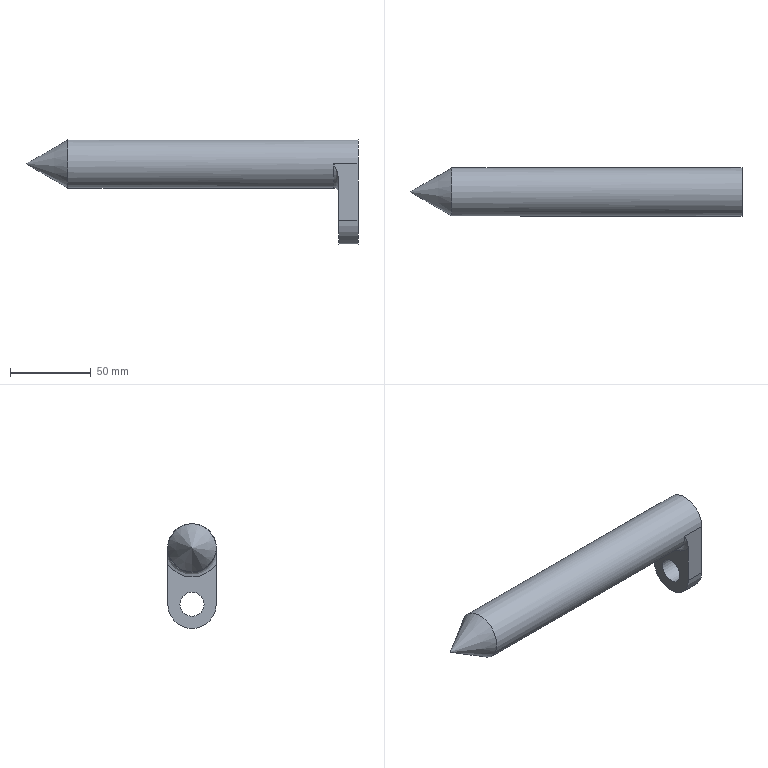Component | NX | CENTRE_HEAD2 | 1 solid | 9 faces | box 205.98 x 30 x 65 mm | volume 143914 mm3 | plane 4 | cylinder 3 | cone 1 | torus 1 | commonest cylinder face diameters 30 x2 15 x1
STEP:
#1=CARTESIAN_POINT('',(0.,0.,0.));
#2=DIRECTION('',(0.,0.,1.));
#3=DIRECTION('',(1.,0.,0.));
#4=AXIS2_PLACEMENT_3D('',#1,#2,#3);
#5=CARTESIAN_POINT('',(157.,15.,137.5));
#6=VERTEX_POINT('',#5);
#7=CARTESIAN_POINT('',(157.,-15.,137.5));
#8=VERTEX_POINT('',#7);
#9=CARTESIAN_POINT('',(157.,0.,137.5));
#10=DIRECTION('',(1.,0.,0.));
#11=DIRECTION('',(0.,0.,-1.));
#12=AXIS2_PLACEMENT_3D('',#9,#10,#11);
#13=CIRCLE('',#12,15.);
#14=CARTESIAN_POINT('',(157.,0.,137.5));
#15=DIRECTION('',(1.,0.,0.));
#16=DIRECTION('',(0.,0.,-1.));
#17=AXIS2_PLACEMENT_3D('',#14,#15,#16);
#18=PLANE('',#17);
#19=CARTESIAN_POINT('',(0.,0.));
#20=DIRECTION('',(1.,0.));
#21=AXIS2_PLACEMENT_2D('',#19,#20);
#22=CIRCLE('',#21,15.);
#23=(GEOMETRIC_REPRESENTATION_CONTEXT(2)PARAMETRIC_REPRESENTATION_CONTEXT()REPRESENTATION_CONTEXT('',''));
#24=DEFINITIONAL_REPRESENTATION('',(#22),#23);
#25=PCURVE('',#18,#24);
#26=CARTESIAN_POINT('',(-48.981,0.,137.5));
#27=DIRECTION('',(1.,0.,0.));
#28=DIRECTION('',(0.,0.,-1.));
#29=AXIS2_PLACEMENT_3D('',#26,#27,#28);
#30=CYLINDRICAL_SURFACE('',#29,15.);
#31=CARTESIAN_POINT('',(0.,205.981));
#32=DIRECTION('',(1.,0.));
#33=VECTOR('',#32,1.);
#34=LINE('',#31,#33);
#35=(GEOMETRIC_REPRESENTATION_CONTEXT(2)PARAMETRIC_REPRESENTATION_CONTEXT()REPRESENTATION_CONTEXT('',''));
#36=DEFINITIONAL_REPRESENTATION('',(#34),#35);
#37=PCURVE('',#30,#36);
#38=SURFACE_CURVE('',#13,(#25,#37),.PCURVE_S1.);
#39=EDGE_CURVE('',#6,#8,#38,.T.);
#40=ORIENTED_EDGE('',*,*,#39,.T.);
#41=CARTESIAN_POINT('',(157.,-15.,102.5));
#42=VERTEX_POINT('',#41);
#43=CARTESIAN_POINT('',(157.,-15.,102.5));
#44=DIRECTION('',(0.,0.,1.));
#45=VECTOR('',#44,1.);
#46=LINE('',#43,#45);
#47=CARTESIAN_POINT('',(35.,-15.));
#48=DIRECTION('',(-1.,0.));
#49=VECTOR('',#48,1.);
#50=LINE('',#47,#49);
#51=(GEOMETRIC_REPRESENTATION_CONTEXT(2)PARAMETRIC_REPRESENTATION_CONTEXT()REPRESENTATION_CONTEXT('',''));
#52=DEFINITIONAL_REPRESENTATION('',(#50),#51);
#53=PCURVE('',#18,#52);
#54=CARTESIAN_POINT('',(145.,-15.,102.5));
#55=DIRECTION('',(0.,1.,-0.));
#56=DIRECTION('',(0.,0.,1.));
#57=AXIS2_PLACEMENT_3D('',#54,#55,#56);
#58=PLANE('',#57);
#59=CARTESIAN_POINT('',(0.,12.));
#60=DIRECTION('',(1.,0.));
#61=VECTOR('',#60,1.);
#62=LINE('',#59,#61);
#63=(GEOMETRIC_REPRESENTATION_CONTEXT(2)PARAMETRIC_REPRESENTATION_CONTEXT()REPRESENTATION_CONTEXT('',''));
#64=DEFINITIONAL_REPRESENTATION('',(#62),#63);
#65=PCURVE('',#58,#64);
#66=SURFACE_CURVE('',#46,(#53,#65),.PCURVE_S1.);
#67=EDGE_CURVE('',#42,#8,#66,.T.);
#68=ORIENTED_EDGE('',*,*,#67,.F.);
#69=CARTESIAN_POINT('',(157.,15.,102.5));
#70=VERTEX_POINT('',#69);
#71=CARTESIAN_POINT('',(157.,0.,102.5));
#72=DIRECTION('',(-1.,0.,0.));
#73=DIRECTION('',(0.,1.,0.));
#74=AXIS2_PLACEMENT_3D('',#71,#72,#73);
#75=CIRCLE('',#74,15.);
#76=CARTESIAN_POINT('',(35.,15.));
#77=CARTESIAN_POINT('',(60.981,15.));
#78=CARTESIAN_POINT('',(47.99,-7.5));
#79=CARTESIAN_POINT('',(35.,-30.));
#80=CARTESIAN_POINT('',(22.01,-7.5));
#81=CARTESIAN_POINT('',(9.019,15.));
#82=CARTESIAN_POINT('',(35.,15.));
#83=(BOUNDED_CURVE()B_SPLINE_CURVE(2,(#76,#77,#78,#79,#80,#81,#82),.UNSPECIFIED.,.T.,.F.)B_SPLINE_CURVE_WITH_KNOTS((1,2,2,2,2,1),(-2.094,0.,2.094,4.189,6.283,8.378),.UNSPECIFIED.)CURVE()GEOMETRIC_REPRESENTATION_ITEM()RATIONAL_B_SPLINE_CURVE((1.,0.5,1.,0.5,1.,0.5,1.))REPRESENTATION_ITEM(''));
#84=(GEOMETRIC_REPRESENTATION_CONTEXT(2)PARAMETRIC_REPRESENTATION_CONTEXT()REPRESENTATION_CONTEXT('',''));
#85=DEFINITIONAL_REPRESENTATION('',(#83),#84);
#86=PCURVE('',#18,#85);
#87=CARTESIAN_POINT('',(145.,0.,102.5));
#88=DIRECTION('',(1.,0.,0.));
#89=DIRECTION('',(0.,0.,-1.));
#90=AXIS2_PLACEMENT_3D('',#87,#88,#89);
#91=CYLINDRICAL_SURFACE('',#90,15.);
#92=CARTESIAN_POINT('',(1.571,12.));
#93=DIRECTION('',(-1.,0.));
#94=VECTOR('',#93,1.);
#95=LINE('',#92,#94);
#96=(GEOMETRIC_REPRESENTATION_CONTEXT(2)PARAMETRIC_REPRESENTATION_CONTEXT()REPRESENTATION_CONTEXT('',''));
#97=DEFINITIONAL_REPRESENTATION('',(#95),#96);
#98=PCURVE('',#91,#97);
#99=SURFACE_CURVE('',#75,(#86,#98),.PCURVE_S1.);
#100=EDGE_CURVE('',#70,#42,#99,.T.);
#101=ORIENTED_EDGE('',*,*,#100,.F.);
#102=CARTESIAN_POINT('',(157.,15.,137.5));
#103=DIRECTION('',(0.,0.,-1.));
#104=VECTOR('',#103,1.);
#105=LINE('',#102,#104);
#106=CARTESIAN_POINT('',(0.,15.));
#107=DIRECTION('',(1.,0.));
#108=VECTOR('',#107,1.);
#109=LINE('',#106,#108);
#110=(GEOMETRIC_REPRESENTATION_CONTEXT(2)PARAMETRIC_REPRESENTATION_CONTEXT()REPRESENTATION_CONTEXT('',''));
#111=DEFINITIONAL_REPRESENTATION('',(#109),#110);
#112=PCURVE('',#18,#111);
#113=CARTESIAN_POINT('',(145.,15.,137.5));
#114=DIRECTION('',(0.,-1.,0.));
#115=DIRECTION('',(0.,0.,-1.));
#116=AXIS2_PLACEMENT_3D('',#113,#114,#115);
#117=PLANE('',#116);
#118=CARTESIAN_POINT('',(0.,12.));
#119=DIRECTION('',(1.,0.));
#120=VECTOR('',#119,1.);
#121=LINE('',#118,#120);
#122=(GEOMETRIC_REPRESENTATION_CONTEXT(2)PARAMETRIC_REPRESENTATION_CONTEXT()REPRESENTATION_CONTEXT('',''));
#123=DEFINITIONAL_REPRESENTATION('',(#121),#122);
#124=PCURVE('',#117,#123);
#125=SURFACE_CURVE('',#105,(#112,#124),.PCURVE_S1.);
#126=EDGE_CURVE('',#6,#70,#125,.T.);
#127=ORIENTED_EDGE('',*,*,#126,.F.);
#128=EDGE_LOOP('',(#40,#68,#101,#127));
#129=FACE_BOUND('',#128,.T.);
#130=CARTESIAN_POINT('',(157.,7.5,102.5));
#131=VERTEX_POINT('',#130);
#132=CARTESIAN_POINT('',(157.,0.,102.5));
#133=DIRECTION('',(-1.,0.,0.));
#134=DIRECTION('',(0.,1.,0.));
#135=AXIS2_PLACEMENT_3D('',#132,#133,#134);
#136=CIRCLE('',#135,7.5);
#137=CARTESIAN_POINT('',(35.,7.5));
#138=CARTESIAN_POINT('',(47.99,7.5));
#139=CARTESIAN_POINT('',(41.495,-3.75));
#140=CARTESIAN_POINT('',(35.,-15.));
#141=CARTESIAN_POINT('',(28.505,-3.75));
#142=CARTESIAN_POINT('',(22.01,7.5));
#143=CARTESIAN_POINT('',(35.,7.5));
#144=(BOUNDED_CURVE()B_SPLINE_CURVE(2,(#137,#138,#139,#140,#141,#142,#143),.UNSPECIFIED.,.T.,.F.)B_SPLINE_CURVE_WITH_KNOTS((1,2,2,2,2,1),(-2.094,0.,2.094,4.189,6.283,8.378),.UNSPECIFIED.)CURVE()GEOMETRIC_REPRESENTATION_ITEM()RATIONAL_B_SPLINE_CURVE((1.,0.5,1.,0.5,1.,0.5,1.))REPRESENTATION_ITEM(''));
#145=(GEOMETRIC_REPRESENTATION_CONTEXT(2)PARAMETRIC_REPRESENTATION_CONTEXT()REPRESENTATION_CONTEXT('',''));
#146=DEFINITIONAL_REPRESENTATION('',(#144),#145);
#147=PCURVE('',#18,#146);
#148=CARTESIAN_POINT('',(145.,0.,102.5));
#149=DIRECTION('',(1.,0.,0.));
#150=DIRECTION('',(0.,0.,-1.));
#151=AXIS2_PLACEMENT_3D('',#148,#149,#150);
#152=CYLINDRICAL_SURFACE('',#151,7.5);
#153=CARTESIAN_POINT('',(7.854,12.));
#154=DIRECTION('',(-1.,0.));
#155=VECTOR('',#154,1.);
#156=LINE('',#153,#155);
#157=(GEOMETRIC_REPRESENTATION_CONTEXT(2)PARAMETRIC_REPRESENTATION_CONTEXT()REPRESENTATION_CONTEXT('',''));
#158=DEFINITIONAL_REPRESENTATION('',(#156),#157);
#159=PCURVE('',#152,#158);
#160=SURFACE_CURVE('',#136,(#147,#159),.PCURVE_S1.);
#161=EDGE_CURVE('',#131,#131,#160,.T.);
#162=ORIENTED_EDGE('',*,*,#161,.T.);
#163=EDGE_LOOP('',(#162));
#164=FACE_BOUND('',#163,.T.);
#165=ADVANCED_FACE('',(#129,#164),#18,.T.);
#166=CARTESIAN_POINT('',(-48.981,0.,137.5));
#167=VERTEX_POINT('',#166);
#168=CARTESIAN_POINT('',(-23.,0.,122.5));
#169=VERTEX_POINT('',#168);
#170=CARTESIAN_POINT('',(-48.981,0.,137.5));
#171=CARTESIAN_POINT('',(-23.,0.,122.5));
#172=B_SPLINE_CURVE_WITH_KNOTS('',1,(#170,#171),.UNSPECIFIED.,.F.,.F.,(2,2),(-30.,0.),.PIECEWISE_BEZIER_KNOTS.);
#173=CARTESIAN_POINT('',(-23.,0.,137.5));
#174=DIRECTION('',(1.,0.,0.));
#175=DIRECTION('',(0.,0.,-1.));
#176=AXIS2_PLACEMENT_3D('',#173,#174,#175);
#177=CONICAL_SURFACE('',#176,15.,0.5236);
#178=CARTESIAN_POINT('',(6.283,0.));
#179=DIRECTION('',(0.,1.));
#180=VECTOR('',#179,1.);
#181=LINE('',#178,#180);
#182=(GEOMETRIC_REPRESENTATION_CONTEXT(2)PARAMETRIC_REPRESENTATION_CONTEXT()REPRESENTATION_CONTEXT('',''));
#183=DEFINITIONAL_REPRESENTATION('',(#181),#182);
#184=PCURVE('',#177,#183);
#185=CARTESIAN_POINT('',(0.,0.));
#186=DIRECTION('',(0.,1.));
#187=VECTOR('',#186,1.);
#188=LINE('',#185,#187);
#189=(GEOMETRIC_REPRESENTATION_CONTEXT(2)PARAMETRIC_REPRESENTATION_CONTEXT()REPRESENTATION_CONTEXT('',''));
#190=DEFINITIONAL_REPRESENTATION('',(#188),#189);
#191=PCURVE('',#177,#190);
#192=SEAM_CURVE('',#172,(#184,#191),.PCURVE_S1.);
#193=EDGE_CURVE('',#167,#169,#192,.T.);
#194=ORIENTED_EDGE('',*,*,#193,.T.);
#195=CARTESIAN_POINT('',(-23.,0.,137.5));
#196=DIRECTION('',(1.,0.,0.));
#197=DIRECTION('',(0.,0.,-1.));
#198=AXIS2_PLACEMENT_3D('',#195,#196,#197);
#199=CIRCLE('',#198,15.);
#200=CARTESIAN_POINT('',(0.,0.));
#201=DIRECTION('',(1.,0.));
#202=VECTOR('',#201,1.);
#203=LINE('',#200,#202);
#204=(GEOMETRIC_REPRESENTATION_CONTEXT(2)PARAMETRIC_REPRESENTATION_CONTEXT()REPRESENTATION_CONTEXT('',''));
#205=DEFINITIONAL_REPRESENTATION('',(#203),#204);
#206=PCURVE('',#177,#205);
#207=CARTESIAN_POINT('',(0.,25.981));
#208=DIRECTION('',(1.,0.));
#209=VECTOR('',#208,1.);
#210=LINE('',#207,#209);
#211=(GEOMETRIC_REPRESENTATION_CONTEXT(2)PARAMETRIC_REPRESENTATION_CONTEXT()REPRESENTATION_CONTEXT('',''));
#212=DEFINITIONAL_REPRESENTATION('',(#210),#211);
#213=PCURVE('',#30,#212);
#214=SURFACE_CURVE('',#199,(#206,#213),.PCURVE_S1.);
#215=EDGE_CURVE('',#169,#169,#214,.T.);
#216=ORIENTED_EDGE('',*,*,#215,.F.);
#217=ORIENTED_EDGE('',*,*,#193,.F.);
#218=EDGE_LOOP('',(#194,#216,#217));
#219=FACE_BOUND('',#218,.T.);
#220=ADVANCED_FACE('',(#219),#177,.T.);
#221=CARTESIAN_POINT('',(142.,15.,137.5));
#222=VERTEX_POINT('',#221);
#223=CARTESIAN_POINT('',(145.,15.,137.5));
#224=DIRECTION('',(1.,0.,0.));
#225=VECTOR('',#224,1.);
#226=LINE('',#223,#225);
#227=CARTESIAN_POINT('',(1.571,193.981));
#228=DIRECTION('',(0.,1.));
#229=VECTOR('',#228,1.);
#230=LINE('',#227,#229);
#231=(GEOMETRIC_REPRESENTATION_CONTEXT(2)PARAMETRIC_REPRESENTATION_CONTEXT()REPRESENTATION_CONTEXT('',''));
#232=DEFINITIONAL_REPRESENTATION('',(#230),#231);
#233=PCURVE('',#30,#232);
#234=CARTESIAN_POINT('',(0.,0.));
#235=DIRECTION('',(0.,1.));
#236=VECTOR('',#235,1.);
#237=LINE('',#234,#236);
#238=(GEOMETRIC_REPRESENTATION_CONTEXT(2)PARAMETRIC_REPRESENTATION_CONTEXT()REPRESENTATION_CONTEXT('',''));
#239=DEFINITIONAL_REPRESENTATION('',(#237),#238);
#240=PCURVE('',#117,#239);
#241=SURFACE_CURVE('',#226,(#233,#240),.PCURVE_S1.);
#242=EDGE_CURVE('',#222,#6,#241,.T.);
#243=ORIENTED_EDGE('',*,*,#242,.F.);
#244=CARTESIAN_POINT('',(142.,0.,122.5));
#245=VERTEX_POINT('',#244);
#246=CARTESIAN_POINT('',(142.,0.,137.5));
#247=DIRECTION('',(-1.,0.,0.));
#248=DIRECTION('',(0.,0.,1.));
#249=AXIS2_PLACEMENT_3D('',#246,#247,#248);
#250=CIRCLE('',#249,15.);
#251=CARTESIAN_POINT('',(3.142,190.981));
#252=DIRECTION('',(-1.,0.));
#253=VECTOR('',#252,1.);
#254=LINE('',#251,#253);
#255=(GEOMETRIC_REPRESENTATION_CONTEXT(2)PARAMETRIC_REPRESENTATION_CONTEXT()REPRESENTATION_CONTEXT('',''));
#256=DEFINITIONAL_REPRESENTATION('',(#254),#255);
#257=PCURVE('',#30,#256);
#258=CARTESIAN_POINT('',(142.,0.,137.5));
#259=DIRECTION('',(-1.,0.,0.));
#260=DIRECTION('',(0.,0.,1.));
#261=AXIS2_PLACEMENT_3D('',#258,#259,#260);
#262=TOROIDAL_SURFACE('',#261,18.,3.);
#263=CARTESIAN_POINT('',(0.,3.142));
#264=DIRECTION('',(1.,0.));
#265=VECTOR('',#264,1.);
#266=LINE('',#263,#265);
#267=(GEOMETRIC_REPRESENTATION_CONTEXT(2)PARAMETRIC_REPRESENTATION_CONTEXT()REPRESENTATION_CONTEXT('',''));
#268=DEFINITIONAL_REPRESENTATION('',(#266),#267);
#269=PCURVE('',#262,#268);
#270=SURFACE_CURVE('',#250,(#257,#269),.PCURVE_S1.);
#271=EDGE_CURVE('',#222,#245,#270,.T.);
#272=ORIENTED_EDGE('',*,*,#271,.T.);
#273=CARTESIAN_POINT('',(-23.,0.,122.5));
#274=CARTESIAN_POINT('',(142.,0.,122.5));
#275=B_SPLINE_CURVE_WITH_KNOTS('',1,(#273,#274),.UNSPECIFIED.,.F.,.F.,(2,2),(25.981,190.981),.PIECEWISE_BEZIER_KNOTS.);
#276=CARTESIAN_POINT('',(0.,0.));
#277=DIRECTION('',(0.,1.));
#278=VECTOR('',#277,1.);
#279=LINE('',#276,#278);
#280=(GEOMETRIC_REPRESENTATION_CONTEXT(2)PARAMETRIC_REPRESENTATION_CONTEXT()REPRESENTATION_CONTEXT('',''));
#281=DEFINITIONAL_REPRESENTATION('',(#279),#280);
#282=PCURVE('',#30,#281);
#283=CARTESIAN_POINT('',(6.283,0.));
#284=DIRECTION('',(0.,1.));
#285=VECTOR('',#284,1.);
#286=LINE('',#283,#285);
#287=(GEOMETRIC_REPRESENTATION_CONTEXT(2)PARAMETRIC_REPRESENTATION_CONTEXT()REPRESENTATION_CONTEXT('',''));
#288=DEFINITIONAL_REPRESENTATION('',(#286),#287);
#289=PCURVE('',#30,#288);
#290=SEAM_CURVE('',#275,(#282,#289),.PCURVE_S1.);
#291=EDGE_CURVE('',#169,#245,#290,.T.);
#292=ORIENTED_EDGE('',*,*,#291,.F.);
#293=ORIENTED_EDGE('',*,*,#215,.T.);
#294=ORIENTED_EDGE('',*,*,#291,.T.);
#295=CARTESIAN_POINT('',(142.,-15.,137.5));
#296=VERTEX_POINT('',#295);
#297=CARTESIAN_POINT('',(142.,0.,137.5));
#298=DIRECTION('',(-1.,0.,0.));
#299=DIRECTION('',(0.,0.,1.));
#300=AXIS2_PLACEMENT_3D('',#297,#298,#299);
#301=CIRCLE('',#300,15.);
#302=CARTESIAN_POINT('',(9.425,190.981));
#303=DIRECTION('',(-1.,0.));
#304=VECTOR('',#303,1.);
#305=LINE('',#302,#304);
#306=(GEOMETRIC_REPRESENTATION_CONTEXT(2)PARAMETRIC_REPRESENTATION_CONTEXT()REPRESENTATION_CONTEXT('',''));
#307=DEFINITIONAL_REPRESENTATION('',(#305),#306);
#308=PCURVE('',#30,#307);
#309=CARTESIAN_POINT('',(0.,3.142));
#310=DIRECTION('',(1.,-0.));
#311=VECTOR('',#310,1.);
#312=LINE('',#309,#311);
#313=(GEOMETRIC_REPRESENTATION_CONTEXT(2)PARAMETRIC_REPRESENTATION_CONTEXT()REPRESENTATION_CONTEXT('',''));
#314=DEFINITIONAL_REPRESENTATION('',(#312),#313);
#315=PCURVE('',#262,#314);
#316=SURFACE_CURVE('',#301,(#308,#315),.PCURVE_S1.);
#317=EDGE_CURVE('',#245,#296,#316,.T.);
#318=ORIENTED_EDGE('',*,*,#317,.T.);
#319=CARTESIAN_POINT('',(145.,-15.,137.5));
#320=DIRECTION('',(1.,0.,0.));
#321=VECTOR('',#320,1.);
#322=LINE('',#319,#321);
#323=CARTESIAN_POINT('',(4.712,193.981));
#324=DIRECTION('',(0.,1.));
#325=VECTOR('',#324,1.);
#326=LINE('',#323,#325);
#327=(GEOMETRIC_REPRESENTATION_CONTEXT(2)PARAMETRIC_REPRESENTATION_CONTEXT()REPRESENTATION_CONTEXT('',''));
#328=DEFINITIONAL_REPRESENTATION('',(#326),#327);
#329=PCURVE('',#30,#328);
#330=CARTESIAN_POINT('',(35.,0.));
#331=DIRECTION('',(0.,1.));
#332=VECTOR('',#331,1.);
#333=LINE('',#330,#332);
#334=(GEOMETRIC_REPRESENTATION_CONTEXT(2)PARAMETRIC_REPRESENTATION_CONTEXT()REPRESENTATION_CONTEXT('',''));
#335=DEFINITIONAL_REPRESENTATION('',(#333),#334);
#336=PCURVE('',#58,#335);
#337=SURFACE_CURVE('',#322,(#329,#336),.PCURVE_S1.);
#338=EDGE_CURVE('',#296,#8,#337,.T.);
#339=ORIENTED_EDGE('',*,*,#338,.T.);
#340=ORIENTED_EDGE('',*,*,#39,.F.);
#341=EDGE_LOOP('',(#243,#272,#292,#293,#294,#318,#339,#340));
#342=FACE_BOUND('',#341,.T.);
#343=ADVANCED_FACE('',(#342),#30,.T.);
#344=ORIENTED_EDGE('',*,*,#67,.T.);
#345=ORIENTED_EDGE('',*,*,#338,.F.);
#346=CARTESIAN_POINT('',(145.,-15.,127.55));
#347=VERTEX_POINT('',#346);
#348=CARTESIAN_POINT('',(142.,-15.,137.5));
#349=CARTESIAN_POINT('',(142.709,-15.,135.915));
#350=CARTESIAN_POINT('',(143.428,-15.,134.313));
#351=CARTESIAN_POINT('',(144.566,-15.,131.009));
#352=CARTESIAN_POINT('',(145.,-15.,129.312));
#353=CARTESIAN_POINT('',(145.,-15.,127.55));
#354=B_SPLINE_CURVE_WITH_KNOTS('',3,(#348,#349,#350,#351,#352,#353),.UNSPECIFIED.,.F.,.F.,(4,2,4),(0.,0.5,1.),.UNSPECIFIED.);
#355=CARTESIAN_POINT('',(35.,-3.));
#356=CARTESIAN_POINT('',(33.415,-2.291));
#357=CARTESIAN_POINT('',(31.813,-1.572));
#358=CARTESIAN_POINT('',(28.509,-0.4343));
#359=CARTESIAN_POINT('',(26.812,0.));
#360=CARTESIAN_POINT('',(25.05,0.));
#361=B_SPLINE_CURVE_WITH_KNOTS('',3,(#355,#356,#357,#358,#359,#360),.UNSPECIFIED.,.F.,.F.,(4,2,4),(0.,0.5,1.),.UNSPECIFIED.);
#362=(GEOMETRIC_REPRESENTATION_CONTEXT(2)PARAMETRIC_REPRESENTATION_CONTEXT()REPRESENTATION_CONTEXT('',''));
#363=DEFINITIONAL_REPRESENTATION('',(#361),#362);
#364=PCURVE('',#58,#363);
#365=CARTESIAN_POINT('',(4.712,3.142));
#366=CARTESIAN_POINT('',(4.703,3.163));
#367=CARTESIAN_POINT('',(4.684,3.206));
#368=CARTESIAN_POINT('',(4.655,3.271));
#369=CARTESIAN_POINT('',(4.626,3.336));
#370=CARTESIAN_POINT('',(4.597,3.401));
#371=CARTESIAN_POINT('',(4.568,3.467));
#372=CARTESIAN_POINT('',(4.54,3.532));
#373=CARTESIAN_POINT('',(4.511,3.599));
#374=CARTESIAN_POINT('',(4.483,3.666));
#375=CARTESIAN_POINT('',(4.455,3.733));
#376=CARTESIAN_POINT('',(4.428,3.801));
#377=CARTESIAN_POINT('',(4.4,3.87));
#378=CARTESIAN_POINT('',(4.373,3.94));
#379=CARTESIAN_POINT('',(4.347,4.01));
#380=CARTESIAN_POINT('',(4.32,4.082));
#381=CARTESIAN_POINT('',(4.294,4.155));
#382=CARTESIAN_POINT('',(4.269,4.229));
#383=CARTESIAN_POINT('',(4.244,4.305));
#384=CARTESIAN_POINT('',(4.22,4.382));
#385=CARTESIAN_POINT('',(4.196,4.46));
#386=CARTESIAN_POINT('',(4.172,4.541));
#387=CARTESIAN_POINT('',(4.149,4.625));
#388=CARTESIAN_POINT('',(4.134,4.683));
#389=CARTESIAN_POINT('',(4.127,4.712));
#390=B_SPLINE_CURVE_WITH_KNOTS('',3,(#365,#366,#367,#368,#369,#370,#371,#372,#373,#374,#375,#376,#377,#378,#379,#380,#381,#382,#383,#384,#385,#386,#387,#388,#389),.UNSPECIFIED.,.F.,.F.,(4,1,1,1,1,1,1,1,1,1,1,1,1,1,1,1,1,1,1,1,1,1,4),(0.,0.04545,0.09091,0.1364,0.1818,0.2273,0.2727,0.3182,0.3636,0.4091,0.4545,0.5,0.5455,0.5909,0.6364,0.6818,0.7273,0.7727,0.8182,0.8636,0.9091,0.9545,1.),.QUASI_UNIFORM_KNOTS.);
#391=(GEOMETRIC_REPRESENTATION_CONTEXT(2)PARAMETRIC_REPRESENTATION_CONTEXT()REPRESENTATION_CONTEXT('',''));
#392=DEFINITIONAL_REPRESENTATION('',(#390),#391);
#393=PCURVE('',#262,#392);
#394=SURFACE_CURVE('',#354,(#364,#393),.PCURVE_S1.);
#395=EDGE_CURVE('',#296,#347,#394,.T.);
#396=ORIENTED_EDGE('',*,*,#395,.T.);
#397=CARTESIAN_POINT('',(145.,-15.,102.5));
#398=VERTEX_POINT('',#397);
#399=CARTESIAN_POINT('',(145.,-15.,102.5));
#400=DIRECTION('',(0.,0.,1.));
#401=VECTOR('',#400,1.);
#402=LINE('',#399,#401);
#403=CARTESIAN_POINT('',(0.,0.));
#404=DIRECTION('',(1.,0.));
#405=VECTOR('',#404,1.);
#406=LINE('',#403,#405);
#407=(GEOMETRIC_REPRESENTATION_CONTEXT(2)PARAMETRIC_REPRESENTATION_CONTEXT()REPRESENTATION_CONTEXT('',''));
#408=DEFINITIONAL_REPRESENTATION('',(#406),#407);
#409=PCURVE('',#58,#408);
#410=CARTESIAN_POINT('',(145.,0.,137.5));
#411=DIRECTION('',(-1.,0.,0.));
#412=DIRECTION('',(0.,0.,1.));
#413=AXIS2_PLACEMENT_3D('',#410,#411,#412);
#414=PLANE('',#413);
#415=CARTESIAN_POINT('',(-35.,-15.));
#416=DIRECTION('',(1.,0.));
#417=VECTOR('',#416,1.);
#418=LINE('',#415,#417);
#419=(GEOMETRIC_REPRESENTATION_CONTEXT(2)PARAMETRIC_REPRESENTATION_CONTEXT()REPRESENTATION_CONTEXT('',''));
#420=DEFINITIONAL_REPRESENTATION('',(#418),#419);
#421=PCURVE('',#414,#420);
#422=SURFACE_CURVE('',#402,(#409,#421),.PCURVE_S1.);
#423=EDGE_CURVE('',#398,#347,#422,.T.);
#424=ORIENTED_EDGE('',*,*,#423,.F.);
#425=CARTESIAN_POINT('',(145.,-15.,102.5));
#426=DIRECTION('',(1.,0.,0.));
#427=VECTOR('',#426,1.);
#428=LINE('',#425,#427);
#429=CARTESIAN_POINT('',(0.,0.));
#430=DIRECTION('',(0.,1.));
#431=VECTOR('',#430,1.);
#432=LINE('',#429,#431);
#433=(GEOMETRIC_REPRESENTATION_CONTEXT(2)PARAMETRIC_REPRESENTATION_CONTEXT()REPRESENTATION_CONTEXT('',''));
#434=DEFINITIONAL_REPRESENTATION('',(#432),#433);
#435=PCURVE('',#58,#434);
#436=CARTESIAN_POINT('',(-1.571,0.));
#437=DIRECTION('',(0.,1.));
#438=VECTOR('',#437,1.);
#439=LINE('',#436,#438);
#440=(GEOMETRIC_REPRESENTATION_CONTEXT(2)PARAMETRIC_REPRESENTATION_CONTEXT()REPRESENTATION_CONTEXT('',''));
#441=DEFINITIONAL_REPRESENTATION('',(#439),#440);
#442=PCURVE('',#91,#441);
#443=SURFACE_CURVE('',#428,(#435,#442),.PCURVE_S1.);
#444=EDGE_CURVE('',#398,#42,#443,.T.);
#445=ORIENTED_EDGE('',*,*,#444,.T.);
#446=EDGE_LOOP('',(#344,#345,#396,#424,#445));
#447=FACE_BOUND('',#446,.T.);
#448=ADVANCED_FACE('',(#447),#58,.F.);
#449=ORIENTED_EDGE('',*,*,#126,.T.);
#450=CARTESIAN_POINT('',(145.,15.,102.5));
#451=VERTEX_POINT('',#450);
#452=CARTESIAN_POINT('',(145.,15.,102.5));
#453=DIRECTION('',(1.,0.,0.));
#454=VECTOR('',#453,1.);
#455=LINE('',#452,#454);
#456=CARTESIAN_POINT('',(35.,0.));
#457=DIRECTION('',(0.,1.));
#458=VECTOR('',#457,1.);
#459=LINE('',#456,#458);
#460=(GEOMETRIC_REPRESENTATION_CONTEXT(2)PARAMETRIC_REPRESENTATION_CONTEXT()REPRESENTATION_CONTEXT('',''));
#461=DEFINITIONAL_REPRESENTATION('',(#459),#460);
#462=PCURVE('',#117,#461);
#463=CARTESIAN_POINT('',(1.571,0.));
#464=DIRECTION('',(0.,1.));
#465=VECTOR('',#464,1.);
#466=LINE('',#463,#465);
#467=(GEOMETRIC_REPRESENTATION_CONTEXT(2)PARAMETRIC_REPRESENTATION_CONTEXT()REPRESENTATION_CONTEXT('',''));
#468=DEFINITIONAL_REPRESENTATION('',(#466),#467);
#469=PCURVE('',#91,#468);
#470=SURFACE_CURVE('',#455,(#462,#469),.PCURVE_S1.);
#471=EDGE_CURVE('',#451,#70,#470,.T.);
#472=ORIENTED_EDGE('',*,*,#471,.F.);
#473=CARTESIAN_POINT('',(145.,15.,127.55));
#474=VERTEX_POINT('',#473);
#475=CARTESIAN_POINT('',(145.,15.,137.5));
#476=DIRECTION('',(0.,0.,-1.));
#477=VECTOR('',#476,1.);
#478=LINE('',#475,#477);
#479=CARTESIAN_POINT('',(0.,0.));
#480=DIRECTION('',(1.,0.));
#481=VECTOR('',#480,1.);
#482=LINE('',#479,#481);
#483=(GEOMETRIC_REPRESENTATION_CONTEXT(2)PARAMETRIC_REPRESENTATION_CONTEXT()REPRESENTATION_CONTEXT('',''));
#484=DEFINITIONAL_REPRESENTATION('',(#482),#483);
#485=PCURVE('',#117,#484);
#486=CARTESIAN_POINT('',(0.,15.));
#487=DIRECTION('',(-1.,0.));
#488=VECTOR('',#487,1.);
#489=LINE('',#486,#488);
#490=(GEOMETRIC_REPRESENTATION_CONTEXT(2)PARAMETRIC_REPRESENTATION_CONTEXT()REPRESENTATION_CONTEXT('',''));
#491=DEFINITIONAL_REPRESENTATION('',(#489),#490);
#492=PCURVE('',#414,#491);
#493=SURFACE_CURVE('',#478,(#485,#492),.PCURVE_S1.);
#494=EDGE_CURVE('',#474,#451,#493,.T.);
#495=ORIENTED_EDGE('',*,*,#494,.F.);
#496=CARTESIAN_POINT('',(145.,15.,127.55));
#497=CARTESIAN_POINT('',(145.,15.,129.312));
#498=CARTESIAN_POINT('',(144.566,15.,131.009));
#499=CARTESIAN_POINT('',(143.428,15.,134.313));
#500=CARTESIAN_POINT('',(142.709,15.,135.915));
#501=CARTESIAN_POINT('',(142.,15.,137.5));
#502=B_SPLINE_CURVE_WITH_KNOTS('',3,(#496,#497,#498,#499,#500,#501),.UNSPECIFIED.,.F.,.F.,(4,2,4),(0.,0.5,1.),.UNSPECIFIED.);
#503=CARTESIAN_POINT('',(9.95,0.));
#504=CARTESIAN_POINT('',(8.188,0.));
#505=CARTESIAN_POINT('',(6.491,-0.4343));
#506=CARTESIAN_POINT('',(3.187,-1.572));
#507=CARTESIAN_POINT('',(1.585,-2.291));
#508=CARTESIAN_POINT('',(0.,-3.));
#509=B_SPLINE_CURVE_WITH_KNOTS('',3,(#503,#504,#505,#506,#507,#508),.UNSPECIFIED.,.F.,.F.,(4,2,4),(0.,0.5,1.),.UNSPECIFIED.);
#510=(GEOMETRIC_REPRESENTATION_CONTEXT(2)PARAMETRIC_REPRESENTATION_CONTEXT()REPRESENTATION_CONTEXT('',''));
#511=DEFINITIONAL_REPRESENTATION('',(#509),#510);
#512=PCURVE('',#117,#511);
#513=CARTESIAN_POINT('',(2.156,4.712));
#514=CARTESIAN_POINT('',(2.149,4.683));
#515=CARTESIAN_POINT('',(2.134,4.625));
#516=CARTESIAN_POINT('',(2.111,4.541));
#517=CARTESIAN_POINT('',(2.088,4.46));
#518=CARTESIAN_POINT('',(2.064,4.382));
#519=CARTESIAN_POINT('',(2.039,4.305));
#520=CARTESIAN_POINT('',(2.014,4.229));
#521=CARTESIAN_POINT('',(1.989,4.155));
#522=CARTESIAN_POINT('',(1.963,4.082));
#523=CARTESIAN_POINT('',(1.937,4.01));
#524=CARTESIAN_POINT('',(1.91,3.94));
#525=CARTESIAN_POINT('',(1.883,3.87));
#526=CARTESIAN_POINT('',(1.856,3.801));
#527=CARTESIAN_POINT('',(1.828,3.733));
#528=CARTESIAN_POINT('',(1.8,3.666));
#529=CARTESIAN_POINT('',(1.772,3.599));
#530=CARTESIAN_POINT('',(1.743,3.532));
#531=CARTESIAN_POINT('',(1.715,3.467));
#532=CARTESIAN_POINT('',(1.686,3.401));
#533=CARTESIAN_POINT('',(1.657,3.336));
#534=CARTESIAN_POINT('',(1.629,3.271));
#535=CARTESIAN_POINT('',(1.6,3.206));
#536=CARTESIAN_POINT('',(1.58,3.163));
#537=CARTESIAN_POINT('',(1.571,3.142));
#538=B_SPLINE_CURVE_WITH_KNOTS('',3,(#513,#514,#515,#516,#517,#518,#519,#520,#521,#522,#523,#524,#525,#526,#527,#528,#529,#530,#531,#532,#533,#534,#535,#536,#537),.UNSPECIFIED.,.F.,.F.,(4,1,1,1,1,1,1,1,1,1,1,1,1,1,1,1,1,1,1,1,1,1,4),(0.,0.04545,0.09091,0.1364,0.1818,0.2273,0.2727,0.3182,0.3636,0.4091,0.4545,0.5,0.5455,0.5909,0.6364,0.6818,0.7273,0.7727,0.8182,0.8636,0.9091,0.9545,1.),.QUASI_UNIFORM_KNOTS.);
#539=(GEOMETRIC_REPRESENTATION_CONTEXT(2)PARAMETRIC_REPRESENTATION_CONTEXT()REPRESENTATION_CONTEXT('',''));
#540=DEFINITIONAL_REPRESENTATION('',(#538),#539);
#541=PCURVE('',#262,#540);
#542=SURFACE_CURVE('',#502,(#512,#541),.PCURVE_S1.);
#543=EDGE_CURVE('',#474,#222,#542,.T.);
#544=ORIENTED_EDGE('',*,*,#543,.T.);
#545=ORIENTED_EDGE('',*,*,#242,.T.);
#546=EDGE_LOOP('',(#449,#472,#495,#544,#545));
#547=FACE_BOUND('',#546,.T.);
#548=ADVANCED_FACE('',(#547),#117,.F.);
#549=ORIENTED_EDGE('',*,*,#100,.T.);
#550=ORIENTED_EDGE('',*,*,#444,.F.);
#551=CARTESIAN_POINT('',(145.,0.,102.5));
#552=DIRECTION('',(-1.,0.,0.));
#553=DIRECTION('',(0.,1.,0.));
#554=AXIS2_PLACEMENT_3D('',#551,#552,#553);
#555=CIRCLE('',#554,15.);
#556=CARTESIAN_POINT('',(1.571,0.));
#557=DIRECTION('',(-1.,0.));
#558=VECTOR('',#557,1.);
#559=LINE('',#556,#558);
#560=(GEOMETRIC_REPRESENTATION_CONTEXT(2)PARAMETRIC_REPRESENTATION_CONTEXT()REPRESENTATION_CONTEXT('',''));
#561=DEFINITIONAL_REPRESENTATION('',(#559),#560);
#562=PCURVE('',#91,#561);
#563=CARTESIAN_POINT('',(-35.,0.));
#564=DIRECTION('',(0.,1.));
#565=AXIS2_PLACEMENT_2D('',#563,#564);
#566=CIRCLE('',#565,15.);
#567=(GEOMETRIC_REPRESENTATION_CONTEXT(2)PARAMETRIC_REPRESENTATION_CONTEXT()REPRESENTATION_CONTEXT('',''));
#568=DEFINITIONAL_REPRESENTATION('',(#566),#567);
#569=PCURVE('',#414,#568);
#570=SURFACE_CURVE('',#555,(#562,#569),.PCURVE_S1.);
#571=EDGE_CURVE('',#451,#398,#570,.T.);
#572=ORIENTED_EDGE('',*,*,#571,.F.);
#573=ORIENTED_EDGE('',*,*,#471,.T.);
#574=EDGE_LOOP('',(#549,#550,#572,#573));
#575=FACE_BOUND('',#574,.T.);
#576=ADVANCED_FACE('',(#575),#91,.T.);
#577=CARTESIAN_POINT('',(145.,7.5,102.5));
#578=VERTEX_POINT('',#577);
#579=CARTESIAN_POINT('',(145.,0.,102.5));
#580=DIRECTION('',(-1.,0.,0.));
#581=DIRECTION('',(0.,1.,0.));
#582=AXIS2_PLACEMENT_3D('',#579,#580,#581);
#583=CIRCLE('',#582,7.5);
#584=CARTESIAN_POINT('',(7.854,0.));
#585=DIRECTION('',(-1.,0.));
#586=VECTOR('',#585,1.);
#587=LINE('',#584,#586);
#588=(GEOMETRIC_REPRESENTATION_CONTEXT(2)PARAMETRIC_REPRESENTATION_CONTEXT()REPRESENTATION_CONTEXT('',''));
#589=DEFINITIONAL_REPRESENTATION('',(#587),#588);
#590=PCURVE('',#152,#589);
#591=CARTESIAN_POINT('',(-35.,0.));
#592=DIRECTION('',(0.,1.));
#593=AXIS2_PLACEMENT_2D('',#591,#592);
#594=CIRCLE('',#593,7.5);
#595=(GEOMETRIC_REPRESENTATION_CONTEXT(2)PARAMETRIC_REPRESENTATION_CONTEXT()REPRESENTATION_CONTEXT('',''));
#596=DEFINITIONAL_REPRESENTATION('',(#594),#595);
#597=PCURVE('',#414,#596);
#598=SURFACE_CURVE('',#583,(#590,#597),.PCURVE_S1.);
#599=EDGE_CURVE('',#578,#578,#598,.T.);
#600=ORIENTED_EDGE('',*,*,#599,.F.);
#601=CARTESIAN_POINT('',(145.,7.5,102.5));
#602=CARTESIAN_POINT('',(157.,7.5,102.5));
#603=B_SPLINE_CURVE_WITH_KNOTS('',1,(#601,#602),.UNSPECIFIED.,.F.,.F.,(2,2),(0.,12.),.PIECEWISE_BEZIER_KNOTS.);
#604=CARTESIAN_POINT('',(7.854,0.));
#605=DIRECTION('',(0.,1.));
#606=VECTOR('',#605,1.);
#607=LINE('',#604,#606);
#608=(GEOMETRIC_REPRESENTATION_CONTEXT(2)PARAMETRIC_REPRESENTATION_CONTEXT()REPRESENTATION_CONTEXT('',''));
#609=DEFINITIONAL_REPRESENTATION('',(#607),#608);
#610=PCURVE('',#152,#609);
#611=CARTESIAN_POINT('',(1.571,0.));
#612=DIRECTION('',(0.,1.));
#613=VECTOR('',#612,1.);
#614=LINE('',#611,#613);
#615=(GEOMETRIC_REPRESENTATION_CONTEXT(2)PARAMETRIC_REPRESENTATION_CONTEXT()REPRESENTATION_CONTEXT('',''));
#616=DEFINITIONAL_REPRESENTATION('',(#614),#615);
#617=PCURVE('',#152,#616);
#618=SEAM_CURVE('',#603,(#610,#617),.PCURVE_S1.);
#619=EDGE_CURVE('',#578,#131,#618,.T.);
#620=ORIENTED_EDGE('',*,*,#619,.T.);
#621=ORIENTED_EDGE('',*,*,#161,.T.);
#622=ORIENTED_EDGE('',*,*,#619,.F.);
#623=EDGE_LOOP('',(#600,#620,#621,#622));
#624=FACE_BOUND('',#623,.F.);
#625=ADVANCED_FACE('',(#624),#152,.F.);
#626=ORIENTED_EDGE('',*,*,#423,.T.);
#627=CARTESIAN_POINT('',(145.,0.,137.5));
#628=DIRECTION('',(1.,0.,0.));
#629=DIRECTION('',(0.,0.,1.));
#630=AXIS2_PLACEMENT_3D('',#627,#628,#629);
#631=CIRCLE('',#630,18.);
#632=CARTESIAN_POINT('',(18.,0.));
#633=CARTESIAN_POINT('',(18.,-31.177));
#634=CARTESIAN_POINT('',(-9.,-15.588));
#635=CARTESIAN_POINT('',(-36.,0.));
#636=CARTESIAN_POINT('',(-9.,15.588));
#637=CARTESIAN_POINT('',(18.,31.177));
#638=CARTESIAN_POINT('',(18.,0.));
#639=(BOUNDED_CURVE()B_SPLINE_CURVE(2,(#632,#633,#634,#635,#636,#637,#638),.UNSPECIFIED.,.T.,.F.)B_SPLINE_CURVE_WITH_KNOTS((1,2,2,2,2,1),(-2.094,0.,2.094,4.189,6.283,8.378),.UNSPECIFIED.)CURVE()GEOMETRIC_REPRESENTATION_ITEM()RATIONAL_B_SPLINE_CURVE((1.,0.5,1.,0.5,1.,0.5,1.))REPRESENTATION_ITEM(''));
#640=(GEOMETRIC_REPRESENTATION_CONTEXT(2)PARAMETRIC_REPRESENTATION_CONTEXT()REPRESENTATION_CONTEXT('',''));
#641=DEFINITIONAL_REPRESENTATION('',(#639),#640);
#642=PCURVE('',#414,#641);
#643=CARTESIAN_POINT('',(6.283,4.712));
#644=DIRECTION('',(-1.,0.));
#645=VECTOR('',#644,1.);
#646=LINE('',#643,#645);
#647=(GEOMETRIC_REPRESENTATION_CONTEXT(2)PARAMETRIC_REPRESENTATION_CONTEXT()REPRESENTATION_CONTEXT('',''));
#648=DEFINITIONAL_REPRESENTATION('',(#646),#647);
#649=PCURVE('',#262,#648);
#650=SURFACE_CURVE('',#631,(#642,#649),.PCURVE_S1.);
#651=EDGE_CURVE('',#347,#474,#650,.T.);
#652=ORIENTED_EDGE('',*,*,#651,.T.);
#653=ORIENTED_EDGE('',*,*,#494,.T.);
#654=ORIENTED_EDGE('',*,*,#571,.T.);
#655=EDGE_LOOP('',(#626,#652,#653,#654));
#656=FACE_BOUND('',#655,.T.);
#657=ORIENTED_EDGE('',*,*,#599,.F.);
#658=EDGE_LOOP('',(#657));
#659=FACE_BOUND('',#658,.T.);
#660=ADVANCED_FACE('',(#656,#659),#414,.T.);
#661=ORIENTED_EDGE('',*,*,#651,.T.);
#662=ORIENTED_EDGE('',*,*,#543,.T.);
#663=ORIENTED_EDGE('',*,*,#271,.T.);
#664=ORIENTED_EDGE('',*,*,#317,.T.);
#665=ORIENTED_EDGE('',*,*,#395,.T.);
#666=EDGE_LOOP('',(#661,#662,#663,#664,#665));
#667=FACE_BOUND('',#666,.F.);
#668=ADVANCED_FACE('',(#667),#262,.F.);
#669=CLOSED_SHELL('',(#165,#220,#343,#448,#548,#576,#625,#660,#668));
#670=MANIFOLD_SOLID_BREP('',#669);
#671=(LENGTH_UNIT()NAMED_UNIT(*)SI_UNIT(.MILLI.,.METRE.));
#672=UNCERTAINTY_MEASURE_WITH_UNIT(LENGTH_MEASURE(0.001),#671,'','');
#673=(NAMED_UNIT(*)PLANE_ANGLE_UNIT()SI_UNIT($,.RADIAN.));
#674=(NAMED_UNIT(*)SI_UNIT($,.STERADIAN.)SOLID_ANGLE_UNIT());
#675=(GEOMETRIC_REPRESENTATION_CONTEXT(3)GLOBAL_UNCERTAINTY_ASSIGNED_CONTEXT((#672))GLOBAL_UNIT_ASSIGNED_CONTEXT((#671,#673,#674))REPRESENTATION_CONTEXT('',''));
#676=ADVANCED_BREP_SHAPE_REPRESENTATION('',(#4,#670),#675);